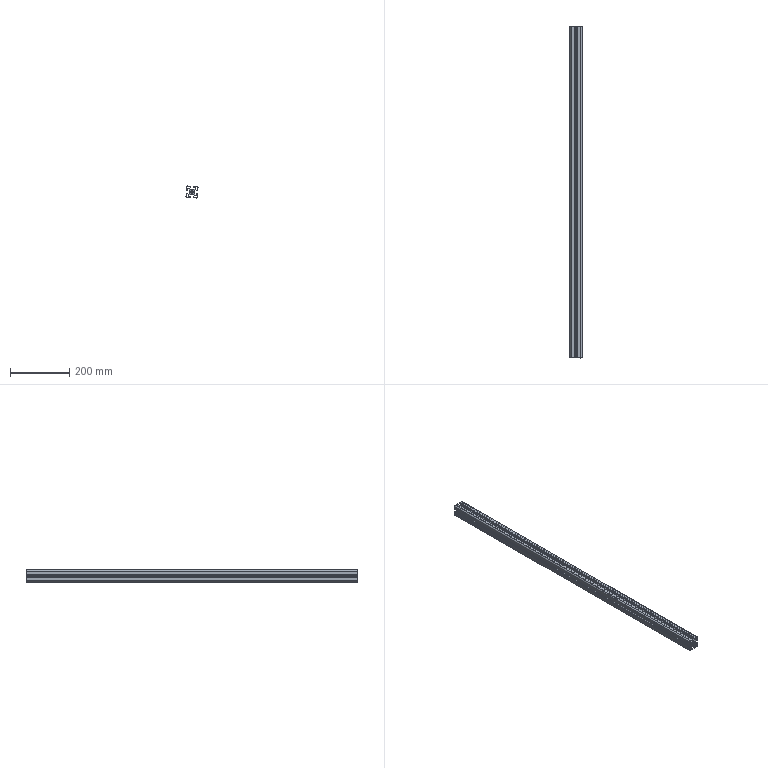Component | SolidWorks | 2012MB0201-1_AUpperRackFrameModule-1_A3007-1 | 1 solid | 147 faces | box 40.73 x 1125 x 40.73 mm | volume 676234 mm3 | plane 117 | cylinder 30 | commonest cylinder face diameters 2 x8 1 x8 6.8 x5 9 x4 5 x4 1.414 x1
build123d program:
from build123d import *

# Parameters (mm, degrees)
BOSS_EXTRUDE1_DEPTH = 1125


with BuildPart() as part:
    # Sketch1 → Boss-Extrude1 (new body)
    with BuildSketch(Plane.XY):
        with BuildLine():
            Line((-19, -4.1), (-19, -5.1))
            Line((-19, -5.1), (-20, -5.1))
            Line((-20, -5.1), (-20, -15.5))
            ThreePointArc((-20, -15.5), (-18.681, -18.682), (-15.499, -20))
            Line((-15.499, -20), (-5.099, -20))
            Line((-5.099, -20), (-5.099, -19))
            Line((-5.099, -19), (-4.099, -19))
            Line((-4.099, -19), (-4.099, -15.5))
            Line((-4.099, -15.5), (-6.599, -15.5))
            Line((-6.599, -15.5), (-6.599, -16.5))
            ThreePointArc((-6.599, -16.5), (-6.892, -17.207), (-7.599, -17.5))
            Line((-7.599, -17.5), (-9.8, -17.5))
            ThreePointArc((-9.8, -17.5), (-10.153, -17.354), (-10.3, -17))
            Line((-10.3, -17), (-10.3, -11.997))
            Line((-10.3, -11.997), (-5.902, -7.6))
            Line((-5.902, -7.6), (-0.5195, -7.6))
            Line((-0.5195, -7.6), (0.0005, -7.3))
            Line((0.0005, -7.3), (0.5195, -7.6))
            Line((0.5195, -7.6), (5.904, -7.6))
            Line((5.904, -7.6), (10.3, -11.997))
            Line((10.3, -11.997), (10.3, -17))
            ThreePointArc((10.3, -17), (10.154, -17.354), (9.8, -17.5))
            Line((9.8, -17.5), (7.601, -17.5))
            ThreePointArc((7.601, -17.5), (6.893, -17.207), (6.601, -16.5))
            Line((6.601, -16.5), (6.601, -15.5))
            Line((6.601, -15.5), (4.101, -15.5))
            Line((4.101, -15.5), (4.101, -19))
            Line((4.101, -19), (5.101, -19))
            Line((5.101, -19), (5.101, -20))
            Line((5.101, -20), (15.501, -20))
            ThreePointArc((15.501, -20), (18.682, -18.682), (20, -15.5))
            Line((20, -15.5), (20, -5.1))
            Line((20, -5.1), (19, -5.1))
            Line((19, -5.1), (19, -4.1))
            Line((19, -4.1), (15.501, -4.1))
            Line((15.501, -4.1), (15.501, -6.6))
            Line((15.501, -6.6), (16.5, -6.6))
            ThreePointArc((16.5, -6.6), (17.208, -6.893), (17.5, -7.6))
            Line((17.5, -7.6), (17.5, -9.8))
            ThreePointArc((17.5, -9.8), (17.354, -10.154), (17, -10.3))
            Line((17, -10.3), (11.998, -10.3))
            Line((11.998, -10.3), (7.601, -5.903))
            Line((7.601, -5.903), (7.601, -0.5203))
            Line((7.601, -0.5203), (7.301, -0.0003417))
            Line((7.301, -0.0003417), (7.601, 0.5197))
            Line((7.601, 0.5197), (7.601, 5.903))
            Line((7.601, 5.903), (11.998, 10.3))
            Line((11.998, 10.3), (17, 10.3))
            ThreePointArc((17, 10.3), (17.354, 10.153), (17.5, 9.8))
            Line((17.5, 9.8), (17.5, 7.6))
            ThreePointArc((17.5, 7.6), (17.208, 6.893), (16.5, 6.6))
            Line((16.5, 6.6), (15.501, 6.6))
            Line((15.501, 6.6), (15.501, 4.1))
            Line((15.501, 4.1), (19, 4.1))
            Line((19, 4.1), (19, 5.1))
            Line((19, 5.1), (20, 5.1))
            Line((20, 5.1), (20, 15.5))
            ThreePointArc((20, 15.5), (18.682, 18.682), (15.501, 20))
            Line((15.501, 20), (5.101, 20))
            Line((5.101, 20), (5.101, 19))
            Line((5.101, 19), (4.101, 19))
            Line((4.101, 19), (4.101, 15.5))
            Line((4.101, 15.5), (6.601, 15.5))
            ThreePointArc((6.601, 15.5), (6.393, 16), (6.601, 16.5))
            ThreePointArc((6.601, 16.5), (6.893, 17.207), (7.601, 17.5))
            Line((7.601, 17.5), (9.8, 17.5))
            ThreePointArc((9.8, 17.5), (10.154, 17.353), (10.3, 17))
            Line((10.3, 17), (10.3, 11.997))
            Line((10.3, 11.997), (5.904, 7.6))
            Line((5.904, 7.6), (0.5195, 7.6))
            Line((0.5195, 7.6), (0.0005, 7.3))
            Line((0.0005, 7.3), (-0.5195, 7.6))
            Line((-0.5195, 7.6), (-5.902, 7.6))
            Line((-5.902, 7.6), (-10.3, 11.997))
            Line((-10.3, 11.997), (-10.3, 17))
            ThreePointArc((-10.3, 17), (-10.153, 17.353), (-9.8, 17.5))
            Line((-9.8, 17.5), (-7.599, 17.5))
            ThreePointArc((-7.599, 17.5), (-6.892, 17.207), (-6.599, 16.5))
            Line((-6.599, 16.5), (-6.599, 15.5))
            Line((-6.599, 15.5), (-4.099, 15.5))
            Line((-4.099, 15.5), (-4.099, 19))
            Line((-4.099, 19), (-5.099, 19))
            Line((-5.099, 19), (-5.099, 20))
            Line((-5.099, 20), (-15.499, 20))
            ThreePointArc((-15.499, 20), (-18.681, 18.682), (-20, 15.5))
            Line((-20, 15.5), (-20, 5.1))
            Line((-20, 5.1), (-19, 5.1))
            Line((-19, 5.1), (-19, 4.1))
            Line((-19, 4.1), (-15.499, 4.1))
            Line((-15.499, 4.1), (-15.499, 6.6))
            Line((-15.499, 6.6), (-16.5, 6.6))
            ThreePointArc((-16.5, 6.6), (-17.207, 6.893), (-17.5, 7.6))
            Line((-17.5, 7.6), (-17.5, 9.8))
            ThreePointArc((-17.5, 9.8), (-17.353, 10.153), (-17, 10.3))
            Line((-17, 10.3), (-11.996, 10.3))
            Line((-11.996, 10.3), (-7.599, 5.903))
            Line((-7.599, 5.903), (-7.599, 0.5197))
            Line((-7.599, 0.5197), (-7.3, -0.0003417))
            Line((-7.3, -0.0003417), (-7.599, -0.5203))
            Line((-7.599, -0.5203), (-7.599, -5.903))
            Line((-7.599, -5.903), (-11.996, -10.3))
            Line((-11.996, -10.3), (-17, -10.3))
            ThreePointArc((-17, -10.3), (-17.353, -10.154), (-17.5, -9.8))
            Line((-17.5, -9.8), (-17.5, -7.6))
            ThreePointArc((-17.5, -7.6), (-17.207, -6.893), (-16.5, -6.6))
            Line((-16.5, -6.6), (-15.499, -6.6))
            Line((-15.499, -6.6), (-15.499, -4.1))
            Line((-15.499, -4.1), (-19, -4.1))
        make_face()
        with BuildLine():
            Line((15.501, -18), (11.8, -18))
            Line((11.8, -18), (11.8, -11.8))
            Line((11.8, -11.8), (18, -11.8))
            Line((18, -11.8), (18, -15.5))
            ThreePointArc((18, -15.5), (17.268, -17.268), (15.501, -18))
        make_face(mode=Mode.SUBTRACT)
        with BuildLine():
            Line((18, 11.8), (11.8, 11.8))
            Line((11.8, 11.8), (11.8, 18))
            Line((11.8, 18), (15.501, 18))
            ThreePointArc((15.501, 18), (17.268, 17.267), (18, 15.5))
            Line((18, 15.5), (18, 11.8))
        make_face(mode=Mode.SUBTRACT)
        with BuildLine():
            Line((-1.815, -2.875), (-3.004, -4.066))
            Line((-3.004, -4.066), (-4.066, -3.005))
            Line((-4.066, -3.005), (-2.874, -1.815))
            ThreePointArc((-2.874, -1.815), (-3.399, -0.0003417), (-2.874, 1.815))
            Line((-2.874, 1.815), (-4.064, 3.006))
            Line((-4.064, 3.006), (-3.004, 4.066))
            Line((-3.004, 4.066), (-1.815, 2.875))
            ThreePointArc((-1.815, 2.875), (0, 3.399), (1.815, 2.875))
            Line((1.815, 2.875), (3.006, 4.066))
            Line((3.006, 4.066), (4.067, 3.005))
            Line((4.067, 3.005), (2.876, 1.815))
            ThreePointArc((2.876, 1.815), (3.4, -0.0003417), (2.876, -1.815))
            Line((2.876, -1.815), (4.067, -3.005))
            Line((4.067, -3.005), (3.006, -4.066))
            Line((3.006, -4.066), (1.815, -2.875))
            ThreePointArc((1.815, -2.875), (0, -3.4), (-1.815, -2.875))
        make_face(mode=Mode.SUBTRACT)
        with BuildLine():
            Line((-18, -15.5), (-18, -11.8))
            Line((-18, -11.8), (-11.8, -11.8))
            Line((-11.8, -11.8), (-11.8, -18))
            Line((-11.8, -18), (-15.499, -18))
            ThreePointArc((-15.499, -18), (-17.267, -17.268), (-18, -15.5))
        make_face(mode=Mode.SUBTRACT)
        with BuildLine():
            Line((-11.8, 18), (-11.8, 11.8))
            Line((-11.8, 11.8), (-18, 11.8))
            Line((-18, 11.8), (-18, 15.5))
            ThreePointArc((-18, 15.5), (-17.267, 17.267), (-15.499, 18))
            Line((-15.499, 18), (-11.8, 18))
        make_face(mode=Mode.SUBTRACT)
    extrude(amount=-BOSS_EXTRUDE1_DEPTH)


solid = part.part

# Placed as in the assembly
solid = solid.moved(Location((-1784.925, -81.15, -1139.586), (90, 0, -1.371)))